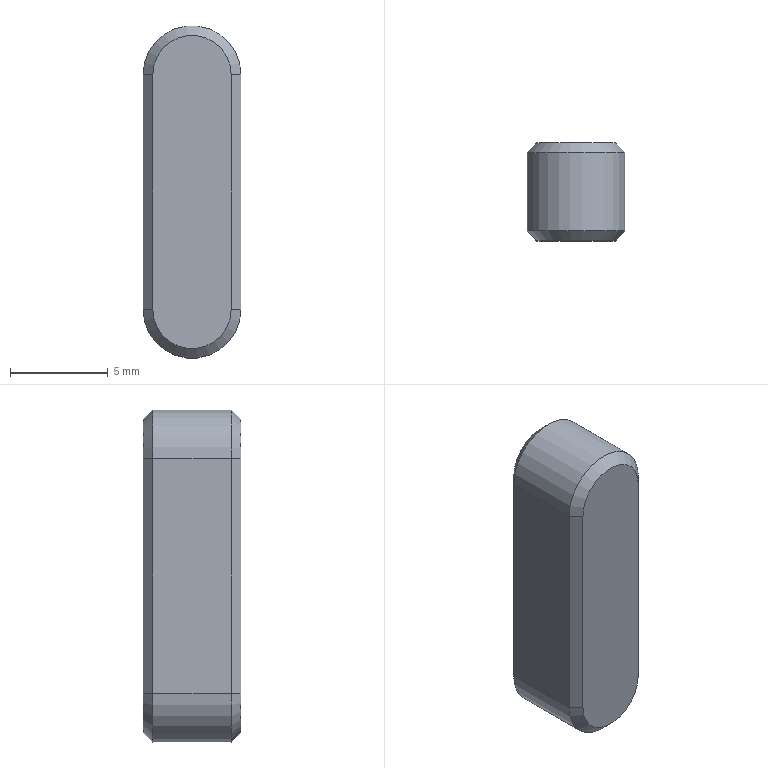Component | SolidWorks | 17x5x5ParallelKey-1 | 1 solid | 14 faces | box 5 x 5 x 17 mm | volume 389 mm3 | plane 8 | cone 4 | cylinder 2 | commonest cylinder face diameters 5 x2 | material AISI 1045 Steel, cold drawn
build123d program:
from build123d import *

# Parameters (mm, degrees)
BOSS_EXTRUDE1_DEPTH = 2.5
CHAMFER1_SIZE       = 0.5


with BuildPart() as part:
    # Sketch1 → Boss-Extrude1 (new, symmetric)
    with BuildSketch(Plane.XY):
        with BuildLine():
            Line((-2.5, -6), (-2.5, 6))
            ThreePointArc((-2.5, 6), (0, 8.5), (2.5, 6))
            Line((2.5, 6), (2.5, -6))
            ThreePointArc((2.5, -6), (0, -8.5), (-2.5, -6))
        make_face()
    extrude(amount=BOSS_EXTRUDE1_DEPTH, both=True)

    # Chamfer1
    chamfer1_edges = [part.edges().sort_by_distance(p)[0] for p in [
        (0, 8.5, 2.5),
        (-2.5, 0, 2.5),
        (0, -8.5, 2.5),
        (-2.5, 0, -2.5),
        (0, 8.5, -2.5),
        (2.5, 0, -2.5),
        (0, -8.5, -2.5),
        (2.5, 0, 2.5),
    ]]
    chamfer(chamfer1_edges, length=CHAMFER1_SIZE)


solid = part.part

# Placed as in the assembly
solid = solid.moved(Location((0, 7.5, 81), (90, 0, 0)))
STEP:
#1=CARTESIAN_POINT('',(-0.09843,0.374,3.425));
#2=VERTEX_POINT('',#1);
#3=CARTESIAN_POINT('',(-0.09843,0.2165,3.425));
#4=VERTEX_POINT('',#3);
#5=CARTESIAN_POINT('',(-0.09843,0.3937,3.425));
#6=DIRECTION('',(0.,-1.,0.));
#7=VECTOR('',#6,39.37);
#8=LINE('',#5,#7);
#9=EDGE_CURVE('',#2,#4,#8,.T.);
#10=ORIENTED_EDGE('',*,*,#9,.T.);
#11=CARTESIAN_POINT('',(0.09843,0.2165,3.425));
#12=VERTEX_POINT('',#11);
#13=CARTESIAN_POINT('',(0.,0.2165,3.425));
#14=DIRECTION('',(-0.,1.,-0.));
#15=DIRECTION('',(1.,0.,0.));
#16=AXIS2_PLACEMENT_3D('',#13,#14,#15);
#17=CIRCLE('',#16,0.09843);
#18=EDGE_CURVE('',#4,#12,#17,.T.);
#19=ORIENTED_EDGE('',*,*,#18,.T.);
#20=CARTESIAN_POINT('',(0.09843,0.374,3.425));
#21=VERTEX_POINT('',#20);
#22=CARTESIAN_POINT('',(0.09843,0.3937,3.425));
#23=DIRECTION('',(0.,-1.,0.));
#24=VECTOR('',#23,39.37);
#25=LINE('',#22,#24);
#26=EDGE_CURVE('',#21,#12,#25,.T.);
#27=ORIENTED_EDGE('',*,*,#26,.F.);
#28=CARTESIAN_POINT('',(0.,0.374,3.425));
#29=DIRECTION('',(0.,-1.,0.));
#30=DIRECTION('',(1.,0.,0.));
#31=AXIS2_PLACEMENT_3D('',#28,#29,#30);
#32=CIRCLE('',#31,0.09843);
#33=EDGE_CURVE('',#21,#2,#32,.T.);
#34=ORIENTED_EDGE('',*,*,#33,.T.);
#35=EDGE_LOOP('',(#10,#19,#27,#34));
#36=FACE_OUTER_BOUND('',#35,.T.);
#37=CARTESIAN_POINT('',(0.,0.3937,3.425));
#38=DIRECTION('',(0.,-1.,0.));
#39=DIRECTION('',(-1.,0.,0.));
#40=AXIS2_PLACEMENT_3D('',#37,#38,#39);
#41=CYLINDRICAL_SURFACE('',#40,0.09843);
#42=ADVANCED_FACE('',(#36),#41,.T.);
#43=ORIENTED_EDGE('',*,*,#26,.T.);
#44=CARTESIAN_POINT('',(0.09843,0.2165,2.953));
#45=VERTEX_POINT('',#44);
#46=CARTESIAN_POINT('',(0.09843,0.2165,3.425));
#47=DIRECTION('',(0.,-0.,-1.));
#48=VECTOR('',#47,39.37);
#49=LINE('',#46,#48);
#50=EDGE_CURVE('',#12,#45,#49,.T.);
#51=ORIENTED_EDGE('',*,*,#50,.T.);
#52=CARTESIAN_POINT('',(0.09843,0.374,2.953));
#53=VERTEX_POINT('',#52);
#54=CARTESIAN_POINT('',(0.09843,0.3937,2.953));
#55=DIRECTION('',(0.,-1.,0.));
#56=VECTOR('',#55,39.37);
#57=LINE('',#54,#56);
#58=EDGE_CURVE('',#53,#45,#57,.T.);
#59=ORIENTED_EDGE('',*,*,#58,.F.);
#60=CARTESIAN_POINT('',(0.09843,0.374,3.425));
#61=DIRECTION('',(-0.,0.,1.));
#62=VECTOR('',#61,39.37);
#63=LINE('',#60,#62);
#64=EDGE_CURVE('',#53,#21,#63,.T.);
#65=ORIENTED_EDGE('',*,*,#64,.T.);
#66=EDGE_LOOP('',(#43,#51,#59,#65));
#67=FACE_OUTER_BOUND('',#66,.T.);
#68=CARTESIAN_POINT('',(0.09843,0.3937,3.425));
#69=DIRECTION('',(-1.,-0.,-0.));
#70=DIRECTION('',(-0.,0.,1.));
#71=AXIS2_PLACEMENT_3D('',#68,#69,#70);
#72=PLANE('',#71);
#73=ADVANCED_FACE('',(#67),#72,.F.);
#74=ORIENTED_EDGE('',*,*,#58,.T.);
#75=CARTESIAN_POINT('',(-0.09843,0.2165,2.953));
#76=VERTEX_POINT('',#75);
#77=CARTESIAN_POINT('',(0.,0.2165,2.953));
#78=DIRECTION('',(-0.,1.,-0.));
#79=DIRECTION('',(1.,0.,0.));
#80=AXIS2_PLACEMENT_3D('',#77,#78,#79);
#81=CIRCLE('',#80,0.09843);
#82=EDGE_CURVE('',#45,#76,#81,.T.);
#83=ORIENTED_EDGE('',*,*,#82,.T.);
#84=CARTESIAN_POINT('',(-0.09843,0.374,2.953));
#85=VERTEX_POINT('',#84);
#86=CARTESIAN_POINT('',(-0.09843,0.3937,2.953));
#87=DIRECTION('',(0.,-1.,0.));
#88=VECTOR('',#87,39.37);
#89=LINE('',#86,#88);
#90=EDGE_CURVE('',#85,#76,#89,.T.);
#91=ORIENTED_EDGE('',*,*,#90,.F.);
#92=CARTESIAN_POINT('',(0.,0.374,2.953));
#93=DIRECTION('',(0.,-1.,0.));
#94=DIRECTION('',(1.,0.,0.));
#95=AXIS2_PLACEMENT_3D('',#92,#93,#94);
#96=CIRCLE('',#95,0.09843);
#97=EDGE_CURVE('',#85,#53,#96,.T.);
#98=ORIENTED_EDGE('',*,*,#97,.T.);
#99=EDGE_LOOP('',(#74,#83,#91,#98));
#100=FACE_OUTER_BOUND('',#99,.T.);
#101=CARTESIAN_POINT('',(0.,0.3937,2.953));
#102=DIRECTION('',(0.,-1.,0.));
#103=DIRECTION('',(-1.,0.,0.));
#104=AXIS2_PLACEMENT_3D('',#101,#102,#103);
#105=CYLINDRICAL_SURFACE('',#104,0.09843);
#106=ADVANCED_FACE('',(#100),#105,.T.);
#107=ORIENTED_EDGE('',*,*,#90,.T.);
#108=CARTESIAN_POINT('',(-0.09843,0.2165,3.425));
#109=DIRECTION('',(-0.,0.,1.));
#110=VECTOR('',#109,39.37);
#111=LINE('',#108,#110);
#112=EDGE_CURVE('',#76,#4,#111,.T.);
#113=ORIENTED_EDGE('',*,*,#112,.T.);
#114=ORIENTED_EDGE('',*,*,#9,.F.);
#115=CARTESIAN_POINT('',(-0.09843,0.374,2.953));
#116=DIRECTION('',(0.,-0.,-1.));
#117=VECTOR('',#116,39.37);
#118=LINE('',#115,#117);
#119=EDGE_CURVE('',#2,#85,#118,.T.);
#120=ORIENTED_EDGE('',*,*,#119,.T.);
#121=EDGE_LOOP('',(#107,#113,#114,#120));
#122=FACE_OUTER_BOUND('',#121,.T.);
#123=CARTESIAN_POINT('',(-0.09843,0.3937,3.425));
#124=DIRECTION('',(1.,0.,0.));
#125=DIRECTION('',(0.,-0.,-1.));
#126=AXIS2_PLACEMENT_3D('',#123,#124,#125);
#127=PLANE('',#126);
#128=ADVANCED_FACE('',(#122),#127,.F.);
#129=CARTESIAN_POINT('',(0.07874,0.3937,2.953));
#130=VERTEX_POINT('',#129);
#131=CARTESIAN_POINT('',(-0.07874,0.3937,2.953));
#132=VERTEX_POINT('',#131);
#133=CARTESIAN_POINT('',(0.,0.3937,2.953));
#134=DIRECTION('',(-0.,1.,-0.));
#135=DIRECTION('',(1.,0.,0.));
#136=AXIS2_PLACEMENT_3D('',#133,#134,#135);
#137=CIRCLE('',#136,0.07874);
#138=EDGE_CURVE('',#130,#132,#137,.T.);
#139=ORIENTED_EDGE('',*,*,#138,.T.);
#140=CARTESIAN_POINT('',(-0.07874,0.3937,3.425));
#141=VERTEX_POINT('',#140);
#142=CARTESIAN_POINT('',(-0.07874,0.3937,3.425));
#143=DIRECTION('',(-0.,0.,1.));
#144=VECTOR('',#143,39.37);
#145=LINE('',#142,#144);
#146=EDGE_CURVE('',#132,#141,#145,.T.);
#147=ORIENTED_EDGE('',*,*,#146,.T.);
#148=CARTESIAN_POINT('',(0.07874,0.3937,3.425));
#149=VERTEX_POINT('',#148);
#150=CARTESIAN_POINT('',(0.,0.3937,3.425));
#151=DIRECTION('',(-0.,1.,-0.));
#152=DIRECTION('',(1.,0.,0.));
#153=AXIS2_PLACEMENT_3D('',#150,#151,#152);
#154=CIRCLE('',#153,0.07874);
#155=EDGE_CURVE('',#141,#149,#154,.T.);
#156=ORIENTED_EDGE('',*,*,#155,.T.);
#157=CARTESIAN_POINT('',(0.07874,0.3937,2.953));
#158=DIRECTION('',(0.,-0.,-1.));
#159=VECTOR('',#158,39.37);
#160=LINE('',#157,#159);
#161=EDGE_CURVE('',#149,#130,#160,.T.);
#162=ORIENTED_EDGE('',*,*,#161,.T.);
#163=EDGE_LOOP('',(#139,#147,#156,#162));
#164=FACE_OUTER_BOUND('',#163,.T.);
#165=CARTESIAN_POINT('',(0.,0.3937,3.425));
#166=DIRECTION('',(-0.,1.,-0.));
#167=DIRECTION('',(1.,0.,0.));
#168=AXIS2_PLACEMENT_3D('',#165,#166,#167);
#169=PLANE('',#168);
#170=ADVANCED_FACE('',(#164),#169,.T.);
#171=CARTESIAN_POINT('',(-0.07874,0.1969,2.953));
#172=VERTEX_POINT('',#171);
#173=CARTESIAN_POINT('',(0.07874,0.1969,2.953));
#174=VERTEX_POINT('',#173);
#175=CARTESIAN_POINT('',(0.,0.1969,2.953));
#176=DIRECTION('',(0.,-1.,0.));
#177=DIRECTION('',(1.,0.,0.));
#178=AXIS2_PLACEMENT_3D('',#175,#176,#177);
#179=CIRCLE('',#178,0.07874);
#180=EDGE_CURVE('',#172,#174,#179,.T.);
#181=ORIENTED_EDGE('',*,*,#180,.T.);
#182=CARTESIAN_POINT('',(0.07874,0.1969,3.425));
#183=VERTEX_POINT('',#182);
#184=CARTESIAN_POINT('',(0.07874,0.1969,3.425));
#185=DIRECTION('',(-0.,0.,1.));
#186=VECTOR('',#185,39.37);
#187=LINE('',#184,#186);
#188=EDGE_CURVE('',#174,#183,#187,.T.);
#189=ORIENTED_EDGE('',*,*,#188,.T.);
#190=CARTESIAN_POINT('',(-0.07874,0.1969,3.425));
#191=VERTEX_POINT('',#190);
#192=CARTESIAN_POINT('',(0.,0.1969,3.425));
#193=DIRECTION('',(0.,-1.,0.));
#194=DIRECTION('',(1.,0.,0.));
#195=AXIS2_PLACEMENT_3D('',#192,#193,#194);
#196=CIRCLE('',#195,0.07874);
#197=EDGE_CURVE('',#183,#191,#196,.T.);
#198=ORIENTED_EDGE('',*,*,#197,.T.);
#199=CARTESIAN_POINT('',(-0.07874,0.1969,3.425));
#200=DIRECTION('',(0.,-0.,-1.));
#201=VECTOR('',#200,39.37);
#202=LINE('',#199,#201);
#203=EDGE_CURVE('',#191,#172,#202,.T.);
#204=ORIENTED_EDGE('',*,*,#203,.T.);
#205=EDGE_LOOP('',(#181,#189,#198,#204));
#206=FACE_OUTER_BOUND('',#205,.T.);
#207=CARTESIAN_POINT('',(0.,0.1969,3.425));
#208=DIRECTION('',(-0.,1.,-0.));
#209=DIRECTION('',(1.,0.,0.));
#210=AXIS2_PLACEMENT_3D('',#207,#208,#209);
#211=PLANE('',#210);
#212=ADVANCED_FACE('',(#206),#211,.F.);
#213=CARTESIAN_POINT('',(-0.07874,0.1969,2.953));
#214=DIRECTION('',(-0.7071,0.7071,-0.));
#215=VECTOR('',#214,39.37);
#216=LINE('',#213,#215);
#217=EDGE_CURVE('',#172,#76,#216,.T.);
#218=ORIENTED_EDGE('',*,*,#217,.F.);
#219=ORIENTED_EDGE('',*,*,#203,.F.);
#220=CARTESIAN_POINT('',(-0.09843,0.2165,3.425));
#221=DIRECTION('',(0.7071,-0.7071,0.));
#222=VECTOR('',#221,39.37);
#223=LINE('',#220,#222);
#224=EDGE_CURVE('',#4,#191,#223,.T.);
#225=ORIENTED_EDGE('',*,*,#224,.F.);
#226=ORIENTED_EDGE('',*,*,#112,.F.);
#227=EDGE_LOOP('',(#218,#219,#225,#226));
#228=FACE_OUTER_BOUND('',#227,.T.);
#229=CARTESIAN_POINT('',(-0.09843,0.2165,3.425));
#230=DIRECTION('',(0.7071,0.7071,0.));
#231=DIRECTION('',(-0.,0.,1.));
#232=AXIS2_PLACEMENT_3D('',#229,#230,#231);
#233=PLANE('',#232);
#234=ADVANCED_FACE('',(#228),#233,.F.);
#235=ORIENTED_EDGE('',*,*,#224,.T.);
#236=ORIENTED_EDGE('',*,*,#197,.F.);
#237=CARTESIAN_POINT('',(0.09843,0.2165,3.425));
#238=DIRECTION('',(-0.7071,-0.7071,-0.));
#239=VECTOR('',#238,39.37);
#240=LINE('',#237,#239);
#241=EDGE_CURVE('',#12,#183,#240,.T.);
#242=ORIENTED_EDGE('',*,*,#241,.F.);
#243=ORIENTED_EDGE('',*,*,#18,.F.);
#244=EDGE_LOOP('',(#235,#236,#242,#243));
#245=FACE_OUTER_BOUND('',#244,.T.);
#246=CARTESIAN_POINT('',(0.,0.2165,3.425));
#247=DIRECTION('',(-0.,1.,-0.));
#248=DIRECTION('',(1.,0.,0.));
#249=AXIS2_PLACEMENT_3D('',#246,#247,#248);
#250=CONICAL_SURFACE('',#249,0.09843,0.7854);
#251=ADVANCED_FACE('',(#245),#250,.T.);
#252=ORIENTED_EDGE('',*,*,#217,.T.);
#253=ORIENTED_EDGE('',*,*,#82,.F.);
#254=CARTESIAN_POINT('',(0.07874,0.1969,2.953));
#255=DIRECTION('',(0.7071,0.7071,0.));
#256=VECTOR('',#255,39.37);
#257=LINE('',#254,#256);
#258=EDGE_CURVE('',#174,#45,#257,.T.);
#259=ORIENTED_EDGE('',*,*,#258,.F.);
#260=ORIENTED_EDGE('',*,*,#180,.F.);
#261=EDGE_LOOP('',(#252,#253,#259,#260));
#262=FACE_OUTER_BOUND('',#261,.T.);
#263=CARTESIAN_POINT('',(0.,0.2165,2.953));
#264=DIRECTION('',(-0.,1.,-0.));
#265=DIRECTION('',(1.,0.,0.));
#266=AXIS2_PLACEMENT_3D('',#263,#264,#265);
#267=CONICAL_SURFACE('',#266,0.09843,0.7854);
#268=ADVANCED_FACE('',(#262),#267,.T.);
#269=ORIENTED_EDGE('',*,*,#241,.T.);
#270=ORIENTED_EDGE('',*,*,#188,.F.);
#271=ORIENTED_EDGE('',*,*,#258,.T.);
#272=ORIENTED_EDGE('',*,*,#50,.F.);
#273=EDGE_LOOP('',(#269,#270,#271,#272));
#274=FACE_OUTER_BOUND('',#273,.T.);
#275=CARTESIAN_POINT('',(0.09843,0.2165,3.425));
#276=DIRECTION('',(-0.7071,0.7071,-0.));
#277=DIRECTION('',(0.,-0.,-1.));
#278=AXIS2_PLACEMENT_3D('',#275,#276,#277);
#279=PLANE('',#278);
#280=ADVANCED_FACE('',(#274),#279,.F.);
#281=CARTESIAN_POINT('',(0.09843,0.374,3.425));
#282=DIRECTION('',(-0.7071,0.7071,-0.));
#283=VECTOR('',#282,39.37);
#284=LINE('',#281,#283);
#285=EDGE_CURVE('',#21,#149,#284,.T.);
#286=ORIENTED_EDGE('',*,*,#285,.F.);
#287=ORIENTED_EDGE('',*,*,#64,.F.);
#288=CARTESIAN_POINT('',(0.07874,0.3937,2.953));
#289=DIRECTION('',(0.7071,-0.7071,0.));
#290=VECTOR('',#289,39.37);
#291=LINE('',#288,#290);
#292=EDGE_CURVE('',#130,#53,#291,.T.);
#293=ORIENTED_EDGE('',*,*,#292,.F.);
#294=ORIENTED_EDGE('',*,*,#161,.F.);
#295=EDGE_LOOP('',(#286,#287,#293,#294));
#296=FACE_OUTER_BOUND('',#295,.T.);
#297=CARTESIAN_POINT('',(0.07874,0.3937,3.425));
#298=DIRECTION('',(0.7071,0.7071,0.));
#299=DIRECTION('',(-0.,0.,1.));
#300=AXIS2_PLACEMENT_3D('',#297,#298,#299);
#301=PLANE('',#300);
#302=ADVANCED_FACE('',(#296),#301,.T.);
#303=ORIENTED_EDGE('',*,*,#292,.T.);
#304=ORIENTED_EDGE('',*,*,#97,.F.);
#305=CARTESIAN_POINT('',(-0.07874,0.3937,2.953));
#306=DIRECTION('',(-0.7071,-0.7071,-0.));
#307=VECTOR('',#306,39.37);
#308=LINE('',#305,#307);
#309=EDGE_CURVE('',#132,#85,#308,.T.);
#310=ORIENTED_EDGE('',*,*,#309,.F.);
#311=ORIENTED_EDGE('',*,*,#138,.F.);
#312=EDGE_LOOP('',(#303,#304,#310,#311));
#313=FACE_OUTER_BOUND('',#312,.T.);
#314=CARTESIAN_POINT('',(0.,0.3937,2.953));
#315=DIRECTION('',(0.,-1.,0.));
#316=DIRECTION('',(-1.,0.,0.));
#317=AXIS2_PLACEMENT_3D('',#314,#315,#316);
#318=CONICAL_SURFACE('',#317,0.07874,0.7854);
#319=ADVANCED_FACE('',(#313),#318,.T.);
#320=ORIENTED_EDGE('',*,*,#285,.T.);
#321=ORIENTED_EDGE('',*,*,#155,.F.);
#322=CARTESIAN_POINT('',(-0.09843,0.374,3.425));
#323=DIRECTION('',(0.7071,0.7071,0.));
#324=VECTOR('',#323,39.37);
#325=LINE('',#322,#324);
#326=EDGE_CURVE('',#2,#141,#325,.T.);
#327=ORIENTED_EDGE('',*,*,#326,.F.);
#328=ORIENTED_EDGE('',*,*,#33,.F.);
#329=EDGE_LOOP('',(#320,#321,#327,#328));
#330=FACE_OUTER_BOUND('',#329,.T.);
#331=CARTESIAN_POINT('',(0.,0.3937,3.425));
#332=DIRECTION('',(0.,-1.,0.));
#333=DIRECTION('',(-1.,0.,0.));
#334=AXIS2_PLACEMENT_3D('',#331,#332,#333);
#335=CONICAL_SURFACE('',#334,0.07874,0.7854);
#336=ADVANCED_FACE('',(#330),#335,.T.);
#337=ORIENTED_EDGE('',*,*,#309,.T.);
#338=ORIENTED_EDGE('',*,*,#119,.F.);
#339=ORIENTED_EDGE('',*,*,#326,.T.);
#340=ORIENTED_EDGE('',*,*,#146,.F.);
#341=EDGE_LOOP('',(#337,#338,#339,#340));
#342=FACE_OUTER_BOUND('',#341,.T.);
#343=CARTESIAN_POINT('',(-0.07874,0.3937,3.425));
#344=DIRECTION('',(-0.7071,0.7071,-0.));
#345=DIRECTION('',(0.,-0.,-1.));
#346=AXIS2_PLACEMENT_3D('',#343,#344,#345);
#347=PLANE('',#346);
#348=ADVANCED_FACE('',(#342),#347,.T.);
#349=CLOSED_SHELL('',(#42,#73,#106,#128,#170,#212,#234,#251,#268,#280,#302,#319,#336,#348));
#350=MANIFOLD_SOLID_BREP('',#349);
#351=CARTESIAN_POINT('',(0.,0.,0.));
#352=DIRECTION('',(0.,0.,1.));
#353=DIRECTION('',(1.,0.,0.));
#354=AXIS2_PLACEMENT_3D('',#351,#352,#353);
#355=(LENGTH_UNIT()NAMED_UNIT(*)SI_UNIT($,.METRE.));
#356=LENGTH_MEASURE_WITH_UNIT(LENGTH_MEASURE(0.0254),#355);
#357=DIMENSIONAL_EXPONENTS(1.,0.,0.,0.,0.,0.,0.);
#358=(CONVERSION_BASED_UNIT('',#356)LENGTH_UNIT()NAMED_UNIT(#357));
#359=UNCERTAINTY_MEASURE_WITH_UNIT(LENGTH_MEASURE(0.00001),#358,'','');
#360=(NAMED_UNIT(*)PLANE_ANGLE_UNIT()SI_UNIT($,.RADIAN.));
#361=(NAMED_UNIT(*)SI_UNIT($,.STERADIAN.)SOLID_ANGLE_UNIT());
#362=(GEOMETRIC_REPRESENTATION_CONTEXT(3)GLOBAL_UNCERTAINTY_ASSIGNED_CONTEXT((#359))GLOBAL_UNIT_ASSIGNED_CONTEXT((#358,#360,#361))REPRESENTATION_CONTEXT('',''));
#363=ADVANCED_BREP_SHAPE_REPRESENTATION('',(#350,#354),#362);
#364=COLOUR_RGB('',0.7922,0.8196,0.9333);
#365=FILL_AREA_STYLE_COLOUR('',#364);
#366=FILL_AREA_STYLE('',(#365));
#367=SURFACE_STYLE_FILL_AREA(#366);
#368=SURFACE_SIDE_STYLE('',(#367));
#369=SURFACE_STYLE_USAGE(.BOTH.,#368);
#370=PRESENTATION_STYLE_ASSIGNMENT((#369));
#371=STYLED_ITEM('',(#370),#350);
#372=PRESENTATION_LAYER_ASSIGNMENT('','',(#371));
#373=(LENGTH_UNIT()NAMED_UNIT(*)SI_UNIT($,.METRE.));
#374=LENGTH_MEASURE_WITH_UNIT(LENGTH_MEASURE(0.0254),#373);
#375=DIMENSIONAL_EXPONENTS(1.,0.,0.,0.,0.,0.,0.);
#376=(CONVERSION_BASED_UNIT('',#374)LENGTH_UNIT()NAMED_UNIT(#375));
#377=UNCERTAINTY_MEASURE_WITH_UNIT(LENGTH_MEASURE(0.00001),#376,'','');
#378=(NAMED_UNIT(*)PLANE_ANGLE_UNIT()SI_UNIT($,.RADIAN.));
#379=(NAMED_UNIT(*)SI_UNIT($,.STERADIAN.)SOLID_ANGLE_UNIT());
#380=(GEOMETRIC_REPRESENTATION_CONTEXT(3)GLOBAL_UNCERTAINTY_ASSIGNED_CONTEXT((#377))GLOBAL_UNIT_ASSIGNED_CONTEXT((#376,#378,#379))REPRESENTATION_CONTEXT('',''));
#381=MECHANICAL_DESIGN_GEOMETRIC_PRESENTATION_REPRESENTATION('',(#371),#380);